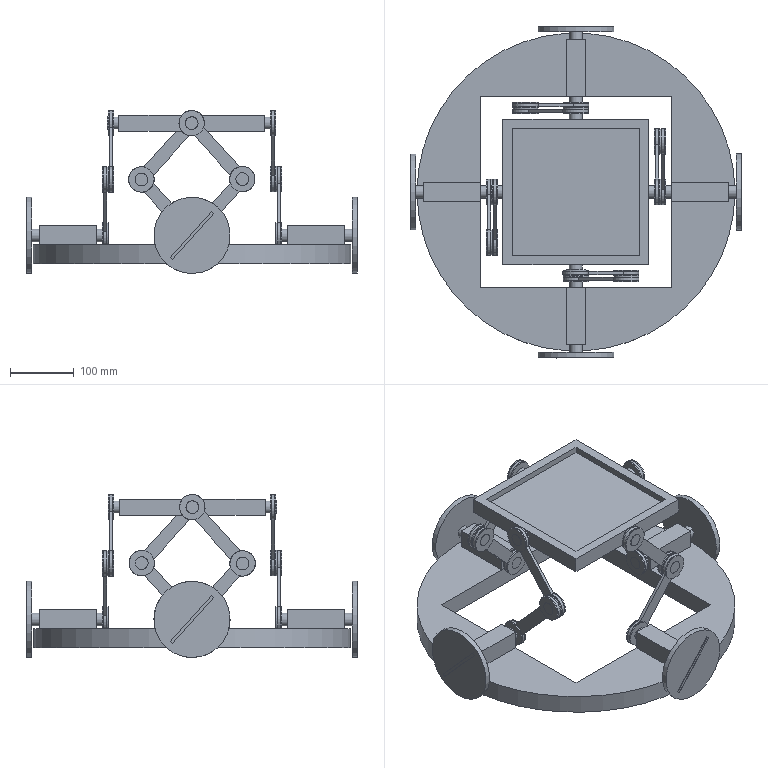Assembly | NX | mm | 18 component files | 58 solids | 302 faces | box 522 x 522 x 256.44 mm | volume 5072128 mm3 | plane 185 | cylinder 117 | commonest cylinder face diameters 20 x64 40 x48 120 x4 500 x1
Bill of materials:
unnamed part 1 | 1 |  | Flat circular disc with a large central square through-opening and four small rectangular blocks standing on the top face, one at the middle of each side of the opening; each block has a round hole running through it parallel to the adjacent opening edge.
unnamed part 2 | 4 |  | Plain solid cylinder with flat ends; length slightly greater than its diameter.
unnamed part 3 | 4 |  | Thin circular disc with a slender cylindrical rod sticking out from the center of one face, at right angles to it; the opposite face seems to have a very thin, slightly smaller-diameter raised layer.
unnamed part 4 | 8 |  | Flat link with a round eye at each end, each with a central through-hole, joined by a straight bar that is narrower and thinner than the eyes.
unnamed part 5 | 1 |  | Square flat plate with a shallow recess on top surrounded by a raised perimeter rim, and a short cylindrical pin sticking out horizontally from the midpoint of each of its four side edges.
Mates:
1. touch align | model3 4 face | model1 1 face
2. fix | model1 1 component
3. distance | model1 1 face | model3 4 face
4. touch align | model3 1 face | model1 1 face
5. touch align | model3 3 face | model1 1 face
6. touch align | model3 2 face | model1 1 face
7. distance | model1 1 face | model3 1 face
8. distance | model1 1 face | model3 3 face
9. distance | model1 1 face | model3 2 face
10. touch align | model2 2 face | model3 1 face
11. distance | model1 1 face | model2 2 face
12. touch align | model2 5 face | model3 4 face
13. touch align | model3 4 face | model2 5 face
14. touch align | model2 1 face | model3 2 face
15. touch align | model2 1 face | model3 2 face
16. touch align | model2 6 face | model3 3 face
17. touch align | model2 6 face | model3 3 face
18. touch align | model5 2 face | model2 6 face
19. touch align | model2 7 face | model5 2 face
20. touch align | model5 2 face | model2 6 face
21. touch align | model2 7 face | model5 2 face
22. touch align | model2 1 face | model5 4 face
23. touch align | model2 3 face | model2 1 face
24. touch align | model5 4 face | model2 1 face
25. touch align | model2 3 face | model5 4 face
26. touch align | model2 5 face | model5 1 face
27. touch align | model5 1 face | model2 4 edge
28. touch align | model2 4 face | model5 1 face
29. touch align | model5 1 face | model2 5 face
30. touch align | model2 2 face | model5 3 face
31. touch align | model5 3 face | model2 8 face
32. touch align | model5 3 face | model2 2 face
33. touch align | model5 3 face | model2 8 face
34. parallel | model3 4 edge | model2 5 edge
35. touch align | model2 4 face | model4 1 face
36. touch align | model2 3 face | model4 1 face
37. touch align | model4 1 face | model2 7 face
38. touch align | model2 8 face | model4 1 face
39. touch align | model2 7 face | model4 1 face
40. touch align | model2 3 face | model4 1 face
41. parallel | model2 6 edge | model3 3 edge